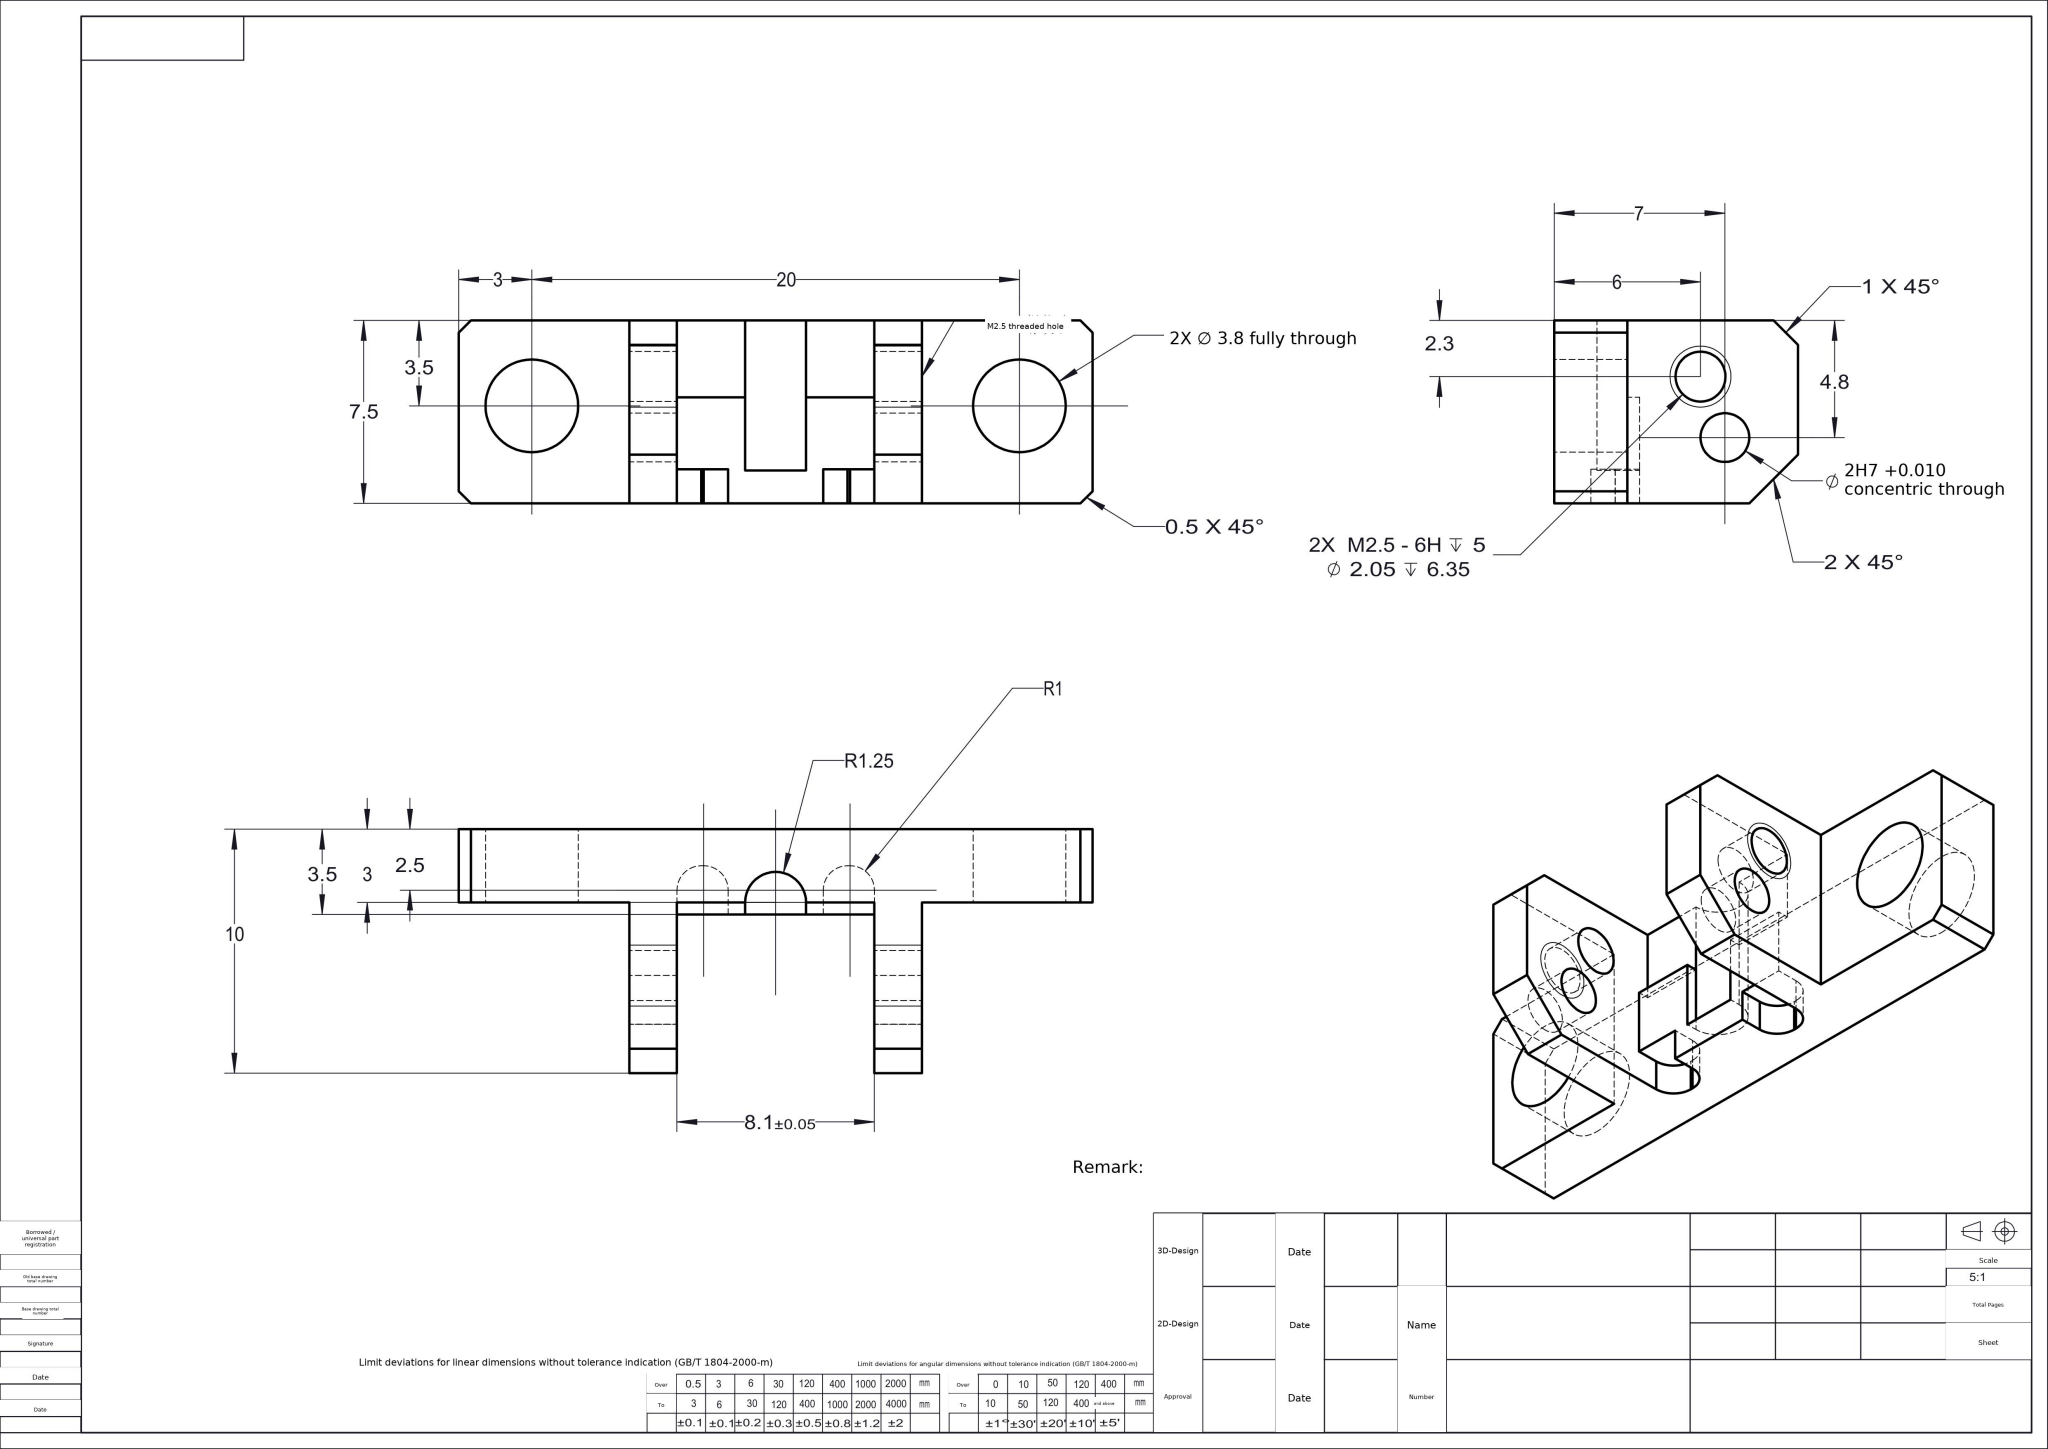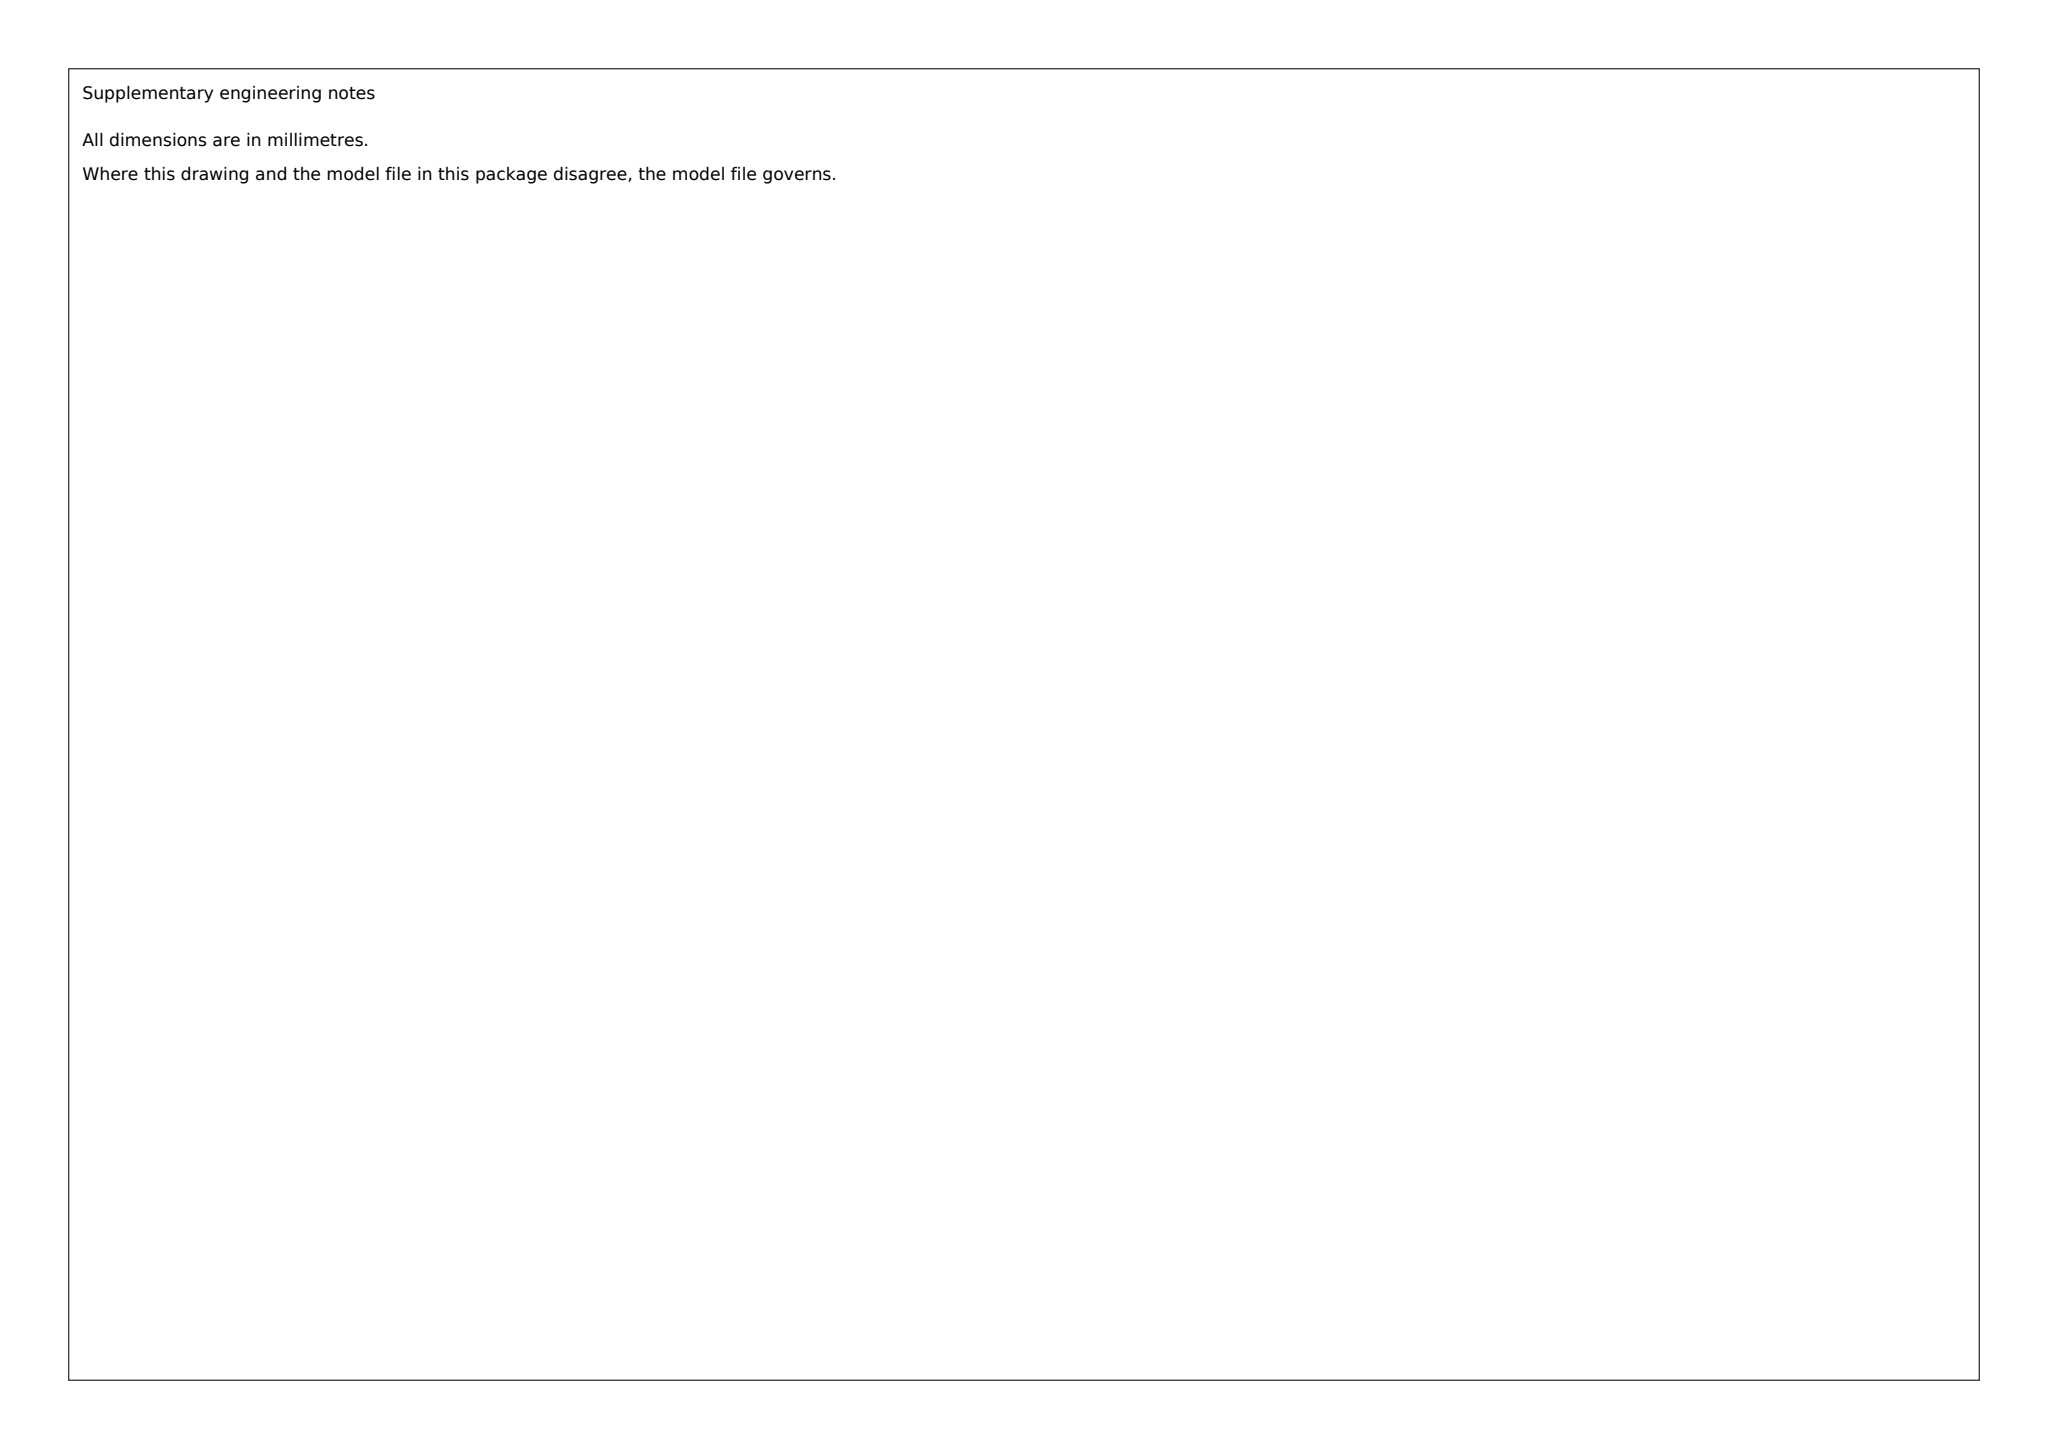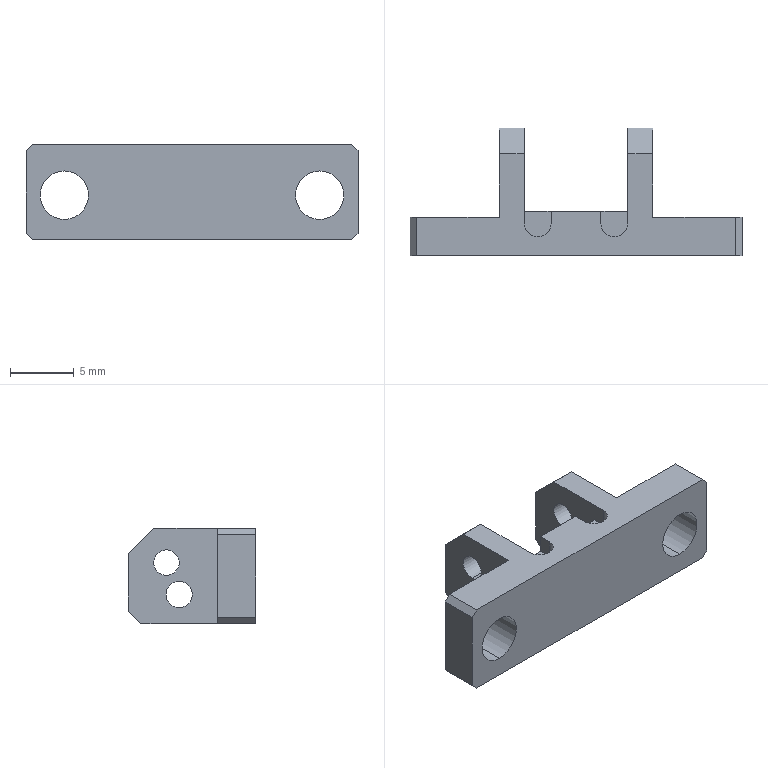Part | SolidWorks | mm | 1 solid | 52 faces | box 26 x 10 x 7.5 mm | volume 674 mm3 | plane 35 | cylinder 17 | commonest cylinder face diameters 2 x8 2.05 x4 3.8 x4 2.5 x1